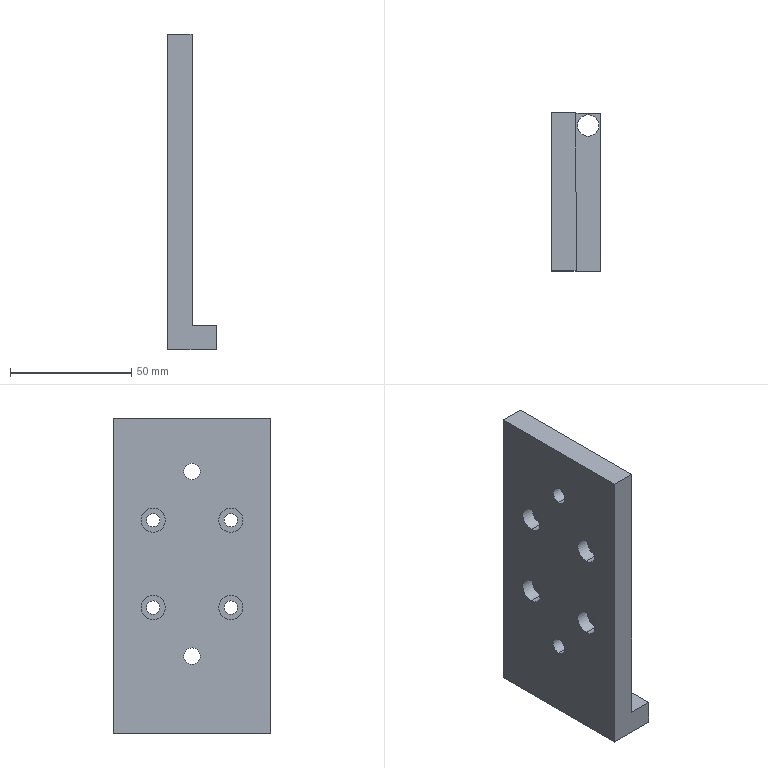Component | SolidWorks | SwingCylinderMountingPlate-1 | 1 solid | 34 faces | box 20.01 x 65 x 130 mm | volume 87532 mm3 | cylinder 22 | plane 12 | commonest cylinder face diameters 10 x8 5.5 x8 6.8 x4 8.8 x2
build123d program:
from build123d import *

# Parameters (mm, degrees)
SKETCH1_W                                       = 120
SKETCH1_H                                       = 65
BOSS_EXTRUDE1_DEPTH                             = 10
M8_TAPPED_HOLE1_D                               = 6.8
M8_TAPPED_HOLE1_DEPTH                           = 19.75
M8_TAPPED_HOLE1_TIP                             = 2.043
M5_HEX_SOCKET_HEAD_CAP_SCREW_CBORE1_D           = 5.5
M5_HEX_SOCKET_HEAD_CAP_SCREW_CBORE1_DEPTH       = 19.75
M5_HEX_SOCKET_HEAD_CAP_SCREW_CBORE1_CBORE_D     = 10
M5_HEX_SOCKET_HEAD_CAP_SCREW_CBORE1_CBORE_DEPTH = 5.4
M5_HEX_SOCKET_HEAD_CAP_SCREW_CBORE1_TIP         = 1.652
SKETCH6_W                                       = 20
SKETCH6_H                                       = 65
BOSS_EXTRUDE2_DEPTH                             = 10
M10X1_25_TAPPED_HOLE1_D                         = 8.8
M10X1_25_TAPPED_HOLE1_DEPTH                     = 23.75
M10X1_25_TAPPED_HOLE1_TIP                       = 2.644


with BuildPart() as part:
    # Sketch1 → Boss-Extrude1 (new body)
    with BuildSketch(Plane.XY):
        Rectangle(SKETCH1_W, SKETCH1_H)
    extrude(amount=BOSS_EXTRUDE1_DEPTH)

    # M8 Tapped Hole1
    with Locations(Plane.XY.offset(10)):
        with Locations((-38, 0), (38, 0)):
            Hole(M8_TAPPED_HOLE1_D / 2, depth=M8_TAPPED_HOLE1_DEPTH)
            with Locations((0, 0, -(M8_TAPPED_HOLE1_DEPTH + M8_TAPPED_HOLE1_TIP / 2))):  # 118° drill point
                Cone(0, M8_TAPPED_HOLE1_D / 2, M8_TAPPED_HOLE1_TIP, mode=Mode.SUBTRACT)

    # M5 Hex Socket Head Cap Screw CBORE1
    with Locations(Plane.XY.offset(10)):
        with Locations((-18, 16), (18, 16), (-18, -16), (18, -16)):
            CounterBoreHole(M5_HEX_SOCKET_HEAD_CAP_SCREW_CBORE1_D / 2, M5_HEX_SOCKET_HEAD_CAP_SCREW_CBORE1_CBORE_D / 2, M5_HEX_SOCKET_HEAD_CAP_SCREW_CBORE1_CBORE_DEPTH, depth=M5_HEX_SOCKET_HEAD_CAP_SCREW_CBORE1_DEPTH)
            with Locations((0, 0, -(M5_HEX_SOCKET_HEAD_CAP_SCREW_CBORE1_DEPTH + M5_HEX_SOCKET_HEAD_CAP_SCREW_CBORE1_TIP / 2))):  # 118° drill point
                Cone(0, M5_HEX_SOCKET_HEAD_CAP_SCREW_CBORE1_D / 2, M5_HEX_SOCKET_HEAD_CAP_SCREW_CBORE1_TIP, mode=Mode.SUBTRACT)

    # Sketch6 → Boss-Extrude2 (add)
    with BuildSketch(Plane.ZY.offset(60)):
        Rectangle(SKETCH6_W, SKETCH6_H)
    extrude(amount=BOSS_EXTRUDE2_DEPTH)

    # M10x1.25 Tapped Hole1
    with Locations(Plane.ZY.offset(70)):
        with Locations((-5, 27.5)):
            Hole(M10X1_25_TAPPED_HOLE1_D / 2, depth=M10X1_25_TAPPED_HOLE1_DEPTH)
            with Locations((0, 0, -(M10X1_25_TAPPED_HOLE1_DEPTH + M10X1_25_TAPPED_HOLE1_TIP / 2))):  # 118° drill point
                Cone(0, M10X1_25_TAPPED_HOLE1_D / 2, M10X1_25_TAPPED_HOLE1_TIP, mode=Mode.SUBTRACT)


solid = part.part

# Placed as in the assembly
solid = solid.moved(Location((1956.163, 3833.759, 1079.241), (0, -90, 0)))
STEP:
#1=CARTESIAN_POINT('',(77.038,152.018,40.128));
#2=VERTEX_POINT('',#1);
#3=CARTESIAN_POINT('',(77.384,152.018,40.128));
#4=VERTEX_POINT('',#3);
#5=CARTESIAN_POINT('',(77.211,152.018,40.128));
#6=DIRECTION('',(-0.,-0.,1.));
#7=DIRECTION('',(1.,0.0001552,0.));
#8=AXIS2_PLACEMENT_3D('',#5,#6,#7);
#9=CIRCLE('',#8,0.1732);
#10=EDGE_CURVE('',#2,#4,#9,.T.);
#11=ORIENTED_EDGE('',*,*,#10,.T.);
#12=CARTESIAN_POINT('',(77.384,152.018,39.734));
#13=VERTEX_POINT('',#12);
#14=CARTESIAN_POINT('',(77.384,152.018,39.734));
#15=DIRECTION('',(0.,0.,-1.));
#16=VECTOR('',#15,39.37);
#17=LINE('',#14,#16);
#18=EDGE_CURVE('',#4,#13,#17,.T.);
#19=ORIENTED_EDGE('',*,*,#18,.T.);
#20=CARTESIAN_POINT('',(77.038,152.018,39.734));
#21=VERTEX_POINT('',#20);
#22=CARTESIAN_POINT('',(77.211,152.018,39.734));
#23=DIRECTION('',(0.,0.,-1.));
#24=DIRECTION('',(-1.,-0.0001552,0.));
#25=AXIS2_PLACEMENT_3D('',#22,#23,#24);
#26=CIRCLE('',#25,0.1732);
#27=EDGE_CURVE('',#13,#21,#26,.T.);
#28=ORIENTED_EDGE('',*,*,#27,.T.);
#29=CARTESIAN_POINT('',(77.038,152.018,39.734));
#30=DIRECTION('',(0.,0.,-1.));
#31=VECTOR('',#30,39.37);
#32=LINE('',#29,#31);
#33=EDGE_CURVE('',#2,#21,#32,.T.);
#34=ORIENTED_EDGE('',*,*,#33,.F.);
#35=EDGE_LOOP('',(#11,#19,#28,#34));
#36=FACE_OUTER_BOUND('',#35,.T.);
#37=CARTESIAN_POINT('',(77.211,152.018,39.734));
#38=DIRECTION('',(0.,0.,-1.));
#39=DIRECTION('',(-1.,-0.0001552,0.));
#40=AXIS2_PLACEMENT_3D('',#37,#38,#39);
#41=CYLINDRICAL_SURFACE('',#40,0.1732);
#42=ADVANCED_FACE('',(#36),#41,.F.);
#43=CARTESIAN_POINT('',(76.833,151.565,41.584));
#44=VERTEX_POINT('',#43);
#45=CARTESIAN_POINT('',(76.833,151.565,41.978));
#46=VERTEX_POINT('',#45);
#47=CARTESIAN_POINT('',(76.833,151.565,41.781));
#48=DIRECTION('',(-1.,-0.0001552,-0.));
#49=DIRECTION('',(0.,0.,1.));
#50=AXIS2_PLACEMENT_3D('',#47,#48,#49);
#51=CIRCLE('',#50,0.1969);
#52=EDGE_CURVE('',#44,#46,#51,.T.);
#53=ORIENTED_EDGE('',*,*,#52,.F.);
#54=CARTESIAN_POINT('',(76.621,151.565,41.584));
#55=VERTEX_POINT('',#54);
#56=CARTESIAN_POINT('',(76.621,151.565,41.584));
#57=DIRECTION('',(-1.,-0.0001552,-0.));
#58=VECTOR('',#57,39.37);
#59=LINE('',#56,#58);
#60=EDGE_CURVE('',#44,#55,#59,.T.);
#61=ORIENTED_EDGE('',*,*,#60,.T.);
#62=CARTESIAN_POINT('',(76.621,151.565,41.978));
#63=VERTEX_POINT('',#62);
#64=CARTESIAN_POINT('',(76.621,151.565,41.781));
#65=DIRECTION('',(-1.,-0.0001552,-0.));
#66=DIRECTION('',(0.,0.,1.));
#67=AXIS2_PLACEMENT_3D('',#64,#65,#66);
#68=CIRCLE('',#67,0.1969);
#69=EDGE_CURVE('',#55,#63,#68,.T.);
#70=ORIENTED_EDGE('',*,*,#69,.T.);
#71=CARTESIAN_POINT('',(76.621,151.565,41.978));
#72=DIRECTION('',(-1.,-0.0001552,-0.));
#73=VECTOR('',#72,39.37);
#74=LINE('',#71,#73);
#75=EDGE_CURVE('',#46,#63,#74,.T.);
#76=ORIENTED_EDGE('',*,*,#75,.F.);
#77=EDGE_LOOP('',(#53,#61,#70,#76));
#78=FACE_OUTER_BOUND('',#77,.T.);
#79=CARTESIAN_POINT('',(76.621,151.565,41.781));
#80=DIRECTION('',(-1.,-0.0001552,-0.));
#81=DIRECTION('',(0.,0.,1.));
#82=AXIS2_PLACEMENT_3D('',#79,#80,#81);
#83=CYLINDRICAL_SURFACE('',#82,0.1969);
#84=ADVANCED_FACE('',(#78),#83,.F.);
#85=CARTESIAN_POINT('',(77.014,151.565,41.673));
#86=VERTEX_POINT('',#85);
#87=CARTESIAN_POINT('',(77.014,151.565,41.889));
#88=VERTEX_POINT('',#87);
#89=CARTESIAN_POINT('',(77.014,151.565,41.781));
#90=DIRECTION('',(-1.,-0.0001552,-0.));
#91=DIRECTION('',(0.,0.,1.));
#92=AXIS2_PLACEMENT_3D('',#89,#90,#91);
#93=CIRCLE('',#92,0.1083);
#94=EDGE_CURVE('',#86,#88,#93,.T.);
#95=ORIENTED_EDGE('',*,*,#94,.F.);
#96=CARTESIAN_POINT('',(76.833,151.565,41.673));
#97=VERTEX_POINT('',#96);
#98=CARTESIAN_POINT('',(76.621,151.565,41.673));
#99=DIRECTION('',(-1.,-0.0001552,-0.));
#100=VECTOR('',#99,39.37);
#101=LINE('',#98,#100);
#102=EDGE_CURVE('',#86,#97,#101,.T.);
#103=ORIENTED_EDGE('',*,*,#102,.T.);
#104=CARTESIAN_POINT('',(76.833,151.565,41.889));
#105=VERTEX_POINT('',#104);
#106=CARTESIAN_POINT('',(76.833,151.565,41.781));
#107=DIRECTION('',(-1.,-0.0001552,-0.));
#108=DIRECTION('',(0.,0.,1.));
#109=AXIS2_PLACEMENT_3D('',#106,#107,#108);
#110=CIRCLE('',#109,0.1083);
#111=EDGE_CURVE('',#97,#105,#110,.T.);
#112=ORIENTED_EDGE('',*,*,#111,.T.);
#113=CARTESIAN_POINT('',(76.621,151.565,41.889));
#114=DIRECTION('',(-1.,-0.0001552,-0.));
#115=VECTOR('',#114,39.37);
#116=LINE('',#113,#115);
#117=EDGE_CURVE('',#88,#105,#116,.T.);
#118=ORIENTED_EDGE('',*,*,#117,.F.);
#119=EDGE_LOOP('',(#95,#103,#112,#118));
#120=FACE_OUTER_BOUND('',#119,.T.);
#121=CARTESIAN_POINT('',(76.621,151.565,41.781));
#122=DIRECTION('',(-1.,-0.0001552,-0.));
#123=DIRECTION('',(0.,0.,1.));
#124=AXIS2_PLACEMENT_3D('',#121,#122,#123);
#125=CYLINDRICAL_SURFACE('',#124,0.1083);
#126=ADVANCED_FACE('',(#120),#125,.F.);
#127=CARTESIAN_POINT('',(76.833,151.565,43.002));
#128=VERTEX_POINT('',#127);
#129=CARTESIAN_POINT('',(76.833,151.565,43.395));
#130=VERTEX_POINT('',#129);
#131=CARTESIAN_POINT('',(76.833,151.565,43.198));
#132=DIRECTION('',(-1.,-0.0001552,-0.));
#133=DIRECTION('',(0.,0.,1.));
#134=AXIS2_PLACEMENT_3D('',#131,#132,#133);
#135=CIRCLE('',#134,0.1969);
#136=EDGE_CURVE('',#128,#130,#135,.T.);
#137=ORIENTED_EDGE('',*,*,#136,.F.);
#138=CARTESIAN_POINT('',(76.621,151.565,43.002));
#139=VERTEX_POINT('',#138);
#140=CARTESIAN_POINT('',(76.621,151.565,43.002));
#141=DIRECTION('',(-1.,-0.0001552,-0.));
#142=VECTOR('',#141,39.37);
#143=LINE('',#140,#142);
#144=EDGE_CURVE('',#128,#139,#143,.T.);
#145=ORIENTED_EDGE('',*,*,#144,.T.);
#146=CARTESIAN_POINT('',(76.621,151.565,43.395));
#147=VERTEX_POINT('',#146);
#148=CARTESIAN_POINT('',(76.621,151.565,43.198));
#149=DIRECTION('',(-1.,-0.0001552,-0.));
#150=DIRECTION('',(0.,0.,1.));
#151=AXIS2_PLACEMENT_3D('',#148,#149,#150);
#152=CIRCLE('',#151,0.1969);
#153=EDGE_CURVE('',#139,#147,#152,.T.);
#154=ORIENTED_EDGE('',*,*,#153,.T.);
#155=CARTESIAN_POINT('',(76.621,151.565,43.395));
#156=DIRECTION('',(-1.,-0.0001552,-0.));
#157=VECTOR('',#156,39.37);
#158=LINE('',#155,#157);
#159=EDGE_CURVE('',#130,#147,#158,.T.);
#160=ORIENTED_EDGE('',*,*,#159,.F.);
#161=EDGE_LOOP('',(#137,#145,#154,#160));
#162=FACE_OUTER_BOUND('',#161,.T.);
#163=CARTESIAN_POINT('',(76.621,151.565,43.198));
#164=DIRECTION('',(-1.,-0.0001552,-0.));
#165=DIRECTION('',(0.,0.,1.));
#166=AXIS2_PLACEMENT_3D('',#163,#164,#165);
#167=CYLINDRICAL_SURFACE('',#166,0.1969);
#168=ADVANCED_FACE('',(#162),#167,.F.);
#169=CARTESIAN_POINT('',(77.014,151.565,43.09));
#170=VERTEX_POINT('',#169);
#171=CARTESIAN_POINT('',(77.014,151.565,43.307));
#172=VERTEX_POINT('',#171);
#173=CARTESIAN_POINT('',(77.014,151.565,43.198));
#174=DIRECTION('',(-1.,-0.0001552,-0.));
#175=DIRECTION('',(0.,0.,1.));
#176=AXIS2_PLACEMENT_3D('',#173,#174,#175);
#177=CIRCLE('',#176,0.1083);
#178=EDGE_CURVE('',#170,#172,#177,.T.);
#179=ORIENTED_EDGE('',*,*,#178,.F.);
#180=CARTESIAN_POINT('',(76.833,151.565,43.09));
#181=VERTEX_POINT('',#180);
#182=CARTESIAN_POINT('',(76.621,151.565,43.09));
#183=DIRECTION('',(-1.,-0.0001552,-0.));
#184=VECTOR('',#183,39.37);
#185=LINE('',#182,#184);
#186=EDGE_CURVE('',#170,#181,#185,.T.);
#187=ORIENTED_EDGE('',*,*,#186,.T.);
#188=CARTESIAN_POINT('',(76.833,151.565,43.307));
#189=VERTEX_POINT('',#188);
#190=CARTESIAN_POINT('',(76.833,151.565,43.198));
#191=DIRECTION('',(-1.,-0.0001552,-0.));
#192=DIRECTION('',(0.,0.,1.));
#193=AXIS2_PLACEMENT_3D('',#190,#191,#192);
#194=CIRCLE('',#193,0.1083);
#195=EDGE_CURVE('',#181,#189,#194,.T.);
#196=ORIENTED_EDGE('',*,*,#195,.T.);
#197=CARTESIAN_POINT('',(76.621,151.565,43.307));
#198=DIRECTION('',(-1.,-0.0001552,-0.));
#199=VECTOR('',#198,39.37);
#200=LINE('',#197,#199);
#201=EDGE_CURVE('',#172,#189,#200,.T.);
#202=ORIENTED_EDGE('',*,*,#201,.F.);
#203=EDGE_LOOP('',(#179,#187,#196,#202));
#204=FACE_OUTER_BOUND('',#203,.T.);
#205=CARTESIAN_POINT('',(76.621,151.565,43.198));
#206=DIRECTION('',(-1.,-0.0001552,-0.));
#207=DIRECTION('',(0.,0.,1.));
#208=AXIS2_PLACEMENT_3D('',#205,#206,#207);
#209=CYLINDRICAL_SURFACE('',#208,0.1083);
#210=ADVANCED_FACE('',(#204),#209,.F.);
#211=CARTESIAN_POINT('',(76.833,150.305,41.584));
#212=VERTEX_POINT('',#211);
#213=CARTESIAN_POINT('',(76.833,150.305,41.978));
#214=VERTEX_POINT('',#213);
#215=CARTESIAN_POINT('',(76.833,150.305,41.781));
#216=DIRECTION('',(-1.,-0.0001552,-0.));
#217=DIRECTION('',(0.,0.,1.));
#218=AXIS2_PLACEMENT_3D('',#215,#216,#217);
#219=CIRCLE('',#218,0.1969);
#220=EDGE_CURVE('',#212,#214,#219,.T.);
#221=ORIENTED_EDGE('',*,*,#220,.F.);
#222=CARTESIAN_POINT('',(76.621,150.305,41.584));
#223=VERTEX_POINT('',#222);
#224=CARTESIAN_POINT('',(76.621,150.305,41.584));
#225=DIRECTION('',(-1.,-0.0001552,-0.));
#226=VECTOR('',#225,39.37);
#227=LINE('',#224,#226);
#228=EDGE_CURVE('',#212,#223,#227,.T.);
#229=ORIENTED_EDGE('',*,*,#228,.T.);
#230=CARTESIAN_POINT('',(76.621,150.305,41.978));
#231=VERTEX_POINT('',#230);
#232=CARTESIAN_POINT('',(76.621,150.305,41.781));
#233=DIRECTION('',(-1.,-0.0001552,-0.));
#234=DIRECTION('',(0.,0.,1.));
#235=AXIS2_PLACEMENT_3D('',#232,#233,#234);
#236=CIRCLE('',#235,0.1969);
#237=EDGE_CURVE('',#223,#231,#236,.T.);
#238=ORIENTED_EDGE('',*,*,#237,.T.);
#239=CARTESIAN_POINT('',(76.621,150.305,41.978));
#240=DIRECTION('',(-1.,-0.0001552,-0.));
#241=VECTOR('',#240,39.37);
#242=LINE('',#239,#241);
#243=EDGE_CURVE('',#214,#231,#242,.T.);
#244=ORIENTED_EDGE('',*,*,#243,.F.);
#245=EDGE_LOOP('',(#221,#229,#238,#244));
#246=FACE_OUTER_BOUND('',#245,.T.);
#247=CARTESIAN_POINT('',(76.621,150.305,41.781));
#248=DIRECTION('',(-1.,-0.0001552,-0.));
#249=DIRECTION('',(0.,0.,1.));
#250=AXIS2_PLACEMENT_3D('',#247,#248,#249);
#251=CYLINDRICAL_SURFACE('',#250,0.1969);
#252=ADVANCED_FACE('',(#246),#251,.F.);
#253=CARTESIAN_POINT('',(77.014,150.305,41.673));
#254=VERTEX_POINT('',#253);
#255=CARTESIAN_POINT('',(77.014,150.305,41.889));
#256=VERTEX_POINT('',#255);
#257=CARTESIAN_POINT('',(77.014,150.305,41.781));
#258=DIRECTION('',(-1.,-0.0001552,-0.));
#259=DIRECTION('',(0.,0.,1.));
#260=AXIS2_PLACEMENT_3D('',#257,#258,#259);
#261=CIRCLE('',#260,0.1083);
#262=EDGE_CURVE('',#254,#256,#261,.T.);
#263=ORIENTED_EDGE('',*,*,#262,.F.);
#264=CARTESIAN_POINT('',(76.833,150.305,41.673));
#265=VERTEX_POINT('',#264);
#266=CARTESIAN_POINT('',(76.621,150.305,41.673));
#267=DIRECTION('',(-1.,-0.0001552,-0.));
#268=VECTOR('',#267,39.37);
#269=LINE('',#266,#268);
#270=EDGE_CURVE('',#254,#265,#269,.T.);
#271=ORIENTED_EDGE('',*,*,#270,.T.);
#272=CARTESIAN_POINT('',(76.833,150.305,41.889));
#273=VERTEX_POINT('',#272);
#274=CARTESIAN_POINT('',(76.833,150.305,41.781));
#275=DIRECTION('',(-1.,-0.0001552,-0.));
#276=DIRECTION('',(0.,0.,1.));
#277=AXIS2_PLACEMENT_3D('',#274,#275,#276);
#278=CIRCLE('',#277,0.1083);
#279=EDGE_CURVE('',#265,#273,#278,.T.);
#280=ORIENTED_EDGE('',*,*,#279,.T.);
#281=CARTESIAN_POINT('',(76.621,150.305,41.889));
#282=DIRECTION('',(-1.,-0.0001552,-0.));
#283=VECTOR('',#282,39.37);
#284=LINE('',#281,#283);
#285=EDGE_CURVE('',#256,#273,#284,.T.);
#286=ORIENTED_EDGE('',*,*,#285,.F.);
#287=EDGE_LOOP('',(#263,#271,#280,#286));
#288=FACE_OUTER_BOUND('',#287,.T.);
#289=CARTESIAN_POINT('',(76.621,150.305,41.781));
#290=DIRECTION('',(-1.,-0.0001552,-0.));
#291=DIRECTION('',(0.,0.,1.));
#292=AXIS2_PLACEMENT_3D('',#289,#290,#291);
#293=CYLINDRICAL_SURFACE('',#292,0.1083);
#294=ADVANCED_FACE('',(#288),#293,.F.);
#295=CARTESIAN_POINT('',(76.833,150.305,43.002));
#296=VERTEX_POINT('',#295);
#297=CARTESIAN_POINT('',(76.833,150.305,43.395));
#298=VERTEX_POINT('',#297);
#299=CARTESIAN_POINT('',(76.833,150.305,43.198));
#300=DIRECTION('',(-1.,-0.0001552,-0.));
#301=DIRECTION('',(0.,0.,1.));
#302=AXIS2_PLACEMENT_3D('',#299,#300,#301);
#303=CIRCLE('',#302,0.1969);
#304=EDGE_CURVE('',#296,#298,#303,.T.);
#305=ORIENTED_EDGE('',*,*,#304,.F.);
#306=CARTESIAN_POINT('',(76.621,150.305,43.002));
#307=VERTEX_POINT('',#306);
#308=CARTESIAN_POINT('',(76.621,150.305,43.002));
#309=DIRECTION('',(-1.,-0.0001552,-0.));
#310=VECTOR('',#309,39.37);
#311=LINE('',#308,#310);
#312=EDGE_CURVE('',#296,#307,#311,.T.);
#313=ORIENTED_EDGE('',*,*,#312,.T.);
#314=CARTESIAN_POINT('',(76.621,150.305,43.395));
#315=VERTEX_POINT('',#314);
#316=CARTESIAN_POINT('',(76.621,150.305,43.198));
#317=DIRECTION('',(-1.,-0.0001552,-0.));
#318=DIRECTION('',(0.,0.,1.));
#319=AXIS2_PLACEMENT_3D('',#316,#317,#318);
#320=CIRCLE('',#319,0.1969);
#321=EDGE_CURVE('',#307,#315,#320,.T.);
#322=ORIENTED_EDGE('',*,*,#321,.T.);
#323=CARTESIAN_POINT('',(76.621,150.305,43.395));
#324=DIRECTION('',(-1.,-0.0001552,-0.));
#325=VECTOR('',#324,39.37);
#326=LINE('',#323,#325);
#327=EDGE_CURVE('',#298,#315,#326,.T.);
#328=ORIENTED_EDGE('',*,*,#327,.F.);
#329=EDGE_LOOP('',(#305,#313,#322,#328));
#330=FACE_OUTER_BOUND('',#329,.T.);
#331=CARTESIAN_POINT('',(76.621,150.305,43.198));
#332=DIRECTION('',(-1.,-0.0001552,-0.));
#333=DIRECTION('',(0.,0.,1.));
#334=AXIS2_PLACEMENT_3D('',#331,#332,#333);
#335=CYLINDRICAL_SURFACE('',#334,0.1969);
#336=ADVANCED_FACE('',(#330),#335,.F.);
#337=CARTESIAN_POINT('',(77.014,150.305,43.09));
#338=VERTEX_POINT('',#337);
#339=CARTESIAN_POINT('',(77.014,150.305,43.307));
#340=VERTEX_POINT('',#339);
#341=CARTESIAN_POINT('',(77.014,150.305,43.198));
#342=DIRECTION('',(-1.,-0.0001552,-0.));
#343=DIRECTION('',(0.,0.,1.));
#344=AXIS2_PLACEMENT_3D('',#341,#342,#343);
#345=CIRCLE('',#344,0.1083);
#346=EDGE_CURVE('',#338,#340,#345,.T.);
#347=ORIENTED_EDGE('',*,*,#346,.F.);
#348=CARTESIAN_POINT('',(76.833,150.305,43.09));
#349=VERTEX_POINT('',#348);
#350=CARTESIAN_POINT('',(76.621,150.305,43.09));
#351=DIRECTION('',(-1.,-0.0001552,-0.));
#352=VECTOR('',#351,39.37);
#353=LINE('',#350,#352);
#354=EDGE_CURVE('',#338,#349,#353,.T.);
#355=ORIENTED_EDGE('',*,*,#354,.T.);
#356=CARTESIAN_POINT('',(76.833,150.305,43.307));
#357=VERTEX_POINT('',#356);
#358=CARTESIAN_POINT('',(76.833,150.305,43.198));
#359=DIRECTION('',(-1.,-0.0001552,-0.));
#360=DIRECTION('',(0.,0.,1.));
#361=AXIS2_PLACEMENT_3D('',#358,#359,#360);
#362=CIRCLE('',#361,0.1083);
#363=EDGE_CURVE('',#349,#357,#362,.T.);
#364=ORIENTED_EDGE('',*,*,#363,.T.);
#365=CARTESIAN_POINT('',(76.621,150.305,43.307));
#366=DIRECTION('',(-1.,-0.0001552,-0.));
#367=VECTOR('',#366,39.37);
#368=LINE('',#365,#367);
#369=EDGE_CURVE('',#340,#357,#368,.T.);
#370=ORIENTED_EDGE('',*,*,#369,.F.);
#371=EDGE_LOOP('',(#347,#355,#364,#370));
#372=FACE_OUTER_BOUND('',#371,.T.);
#373=CARTESIAN_POINT('',(76.621,150.305,43.198));
#374=DIRECTION('',(-1.,-0.0001552,-0.));
#375=DIRECTION('',(0.,0.,1.));
#376=AXIS2_PLACEMENT_3D('',#373,#374,#375);
#377=CYLINDRICAL_SURFACE('',#376,0.1083);
#378=ADVANCED_FACE('',(#372),#377,.F.);
#379=CARTESIAN_POINT('',(77.014,150.935,40.86));
#380=VERTEX_POINT('',#379);
#381=CARTESIAN_POINT('',(77.014,150.935,41.128));
#382=VERTEX_POINT('',#381);
#383=CARTESIAN_POINT('',(77.014,150.935,40.994));
#384=DIRECTION('',(-1.,-0.0001552,-0.));
#385=DIRECTION('',(0.,0.,1.));
#386=AXIS2_PLACEMENT_3D('',#383,#384,#385);
#387=CIRCLE('',#386,0.1339);
#388=EDGE_CURVE('',#380,#382,#387,.T.);
#389=ORIENTED_EDGE('',*,*,#388,.F.);
#390=CARTESIAN_POINT('',(76.621,150.935,40.86));
#391=VERTEX_POINT('',#390);
#392=CARTESIAN_POINT('',(76.621,150.935,40.86));
#393=DIRECTION('',(-1.,-0.0001552,-0.));
#394=VECTOR('',#393,39.37);
#395=LINE('',#392,#394);
#396=EDGE_CURVE('',#380,#391,#395,.T.);
#397=ORIENTED_EDGE('',*,*,#396,.T.);
#398=CARTESIAN_POINT('',(76.621,150.935,41.128));
#399=VERTEX_POINT('',#398);
#400=CARTESIAN_POINT('',(76.621,150.935,40.994));
#401=DIRECTION('',(-1.,-0.0001552,-0.));
#402=DIRECTION('',(0.,0.,1.));
#403=AXIS2_PLACEMENT_3D('',#400,#401,#402);
#404=CIRCLE('',#403,0.1339);
#405=EDGE_CURVE('',#391,#399,#404,.T.);
#406=ORIENTED_EDGE('',*,*,#405,.T.);
#407=CARTESIAN_POINT('',(76.621,150.935,41.128));
#408=DIRECTION('',(-1.,-0.0001552,-0.));
#409=VECTOR('',#408,39.37);
#410=LINE('',#407,#409);
#411=EDGE_CURVE('',#382,#399,#410,.T.);
#412=ORIENTED_EDGE('',*,*,#411,.F.);
#413=EDGE_LOOP('',(#389,#397,#406,#412));
#414=FACE_OUTER_BOUND('',#413,.T.);
#415=CARTESIAN_POINT('',(76.621,150.935,40.994));
#416=DIRECTION('',(-1.,-0.0001552,-0.));
#417=DIRECTION('',(0.,0.,1.));
#418=AXIS2_PLACEMENT_3D('',#415,#416,#417);
#419=CYLINDRICAL_SURFACE('',#418,0.1339);
#420=ADVANCED_FACE('',(#414),#419,.F.);
#421=CARTESIAN_POINT('',(77.014,150.935,43.852));
#422=VERTEX_POINT('',#421);
#423=CARTESIAN_POINT('',(77.014,150.935,44.12));
#424=VERTEX_POINT('',#423);
#425=CARTESIAN_POINT('',(77.014,150.935,43.986));
#426=DIRECTION('',(-1.,-0.0001552,-0.));
#427=DIRECTION('',(0.,0.,1.));
#428=AXIS2_PLACEMENT_3D('',#425,#426,#427);
#429=CIRCLE('',#428,0.1339);
#430=EDGE_CURVE('',#422,#424,#429,.T.);
#431=ORIENTED_EDGE('',*,*,#430,.F.);
#432=CARTESIAN_POINT('',(76.621,150.935,43.852));
#433=VERTEX_POINT('',#432);
#434=CARTESIAN_POINT('',(76.621,150.935,43.852));
#435=DIRECTION('',(-1.,-0.0001552,-0.));
#436=VECTOR('',#435,39.37);
#437=LINE('',#434,#436);
#438=EDGE_CURVE('',#422,#433,#437,.T.);
#439=ORIENTED_EDGE('',*,*,#438,.T.);
#440=CARTESIAN_POINT('',(76.621,150.935,44.12));
#441=VERTEX_POINT('',#440);
#442=CARTESIAN_POINT('',(76.621,150.935,43.986));
#443=DIRECTION('',(-1.,-0.0001552,-0.));
#444=DIRECTION('',(0.,0.,1.));
#445=AXIS2_PLACEMENT_3D('',#442,#443,#444);
#446=CIRCLE('',#445,0.1339);
#447=EDGE_CURVE('',#433,#441,#446,.T.);
#448=ORIENTED_EDGE('',*,*,#447,.T.);
#449=CARTESIAN_POINT('',(76.621,150.935,44.12));
#450=DIRECTION('',(-1.,-0.0001552,-0.));
#451=VECTOR('',#450,39.37);
#452=LINE('',#449,#451);
#453=EDGE_CURVE('',#424,#441,#452,.T.);
#454=ORIENTED_EDGE('',*,*,#453,.F.);
#455=EDGE_LOOP('',(#431,#439,#448,#454));
#456=FACE_OUTER_BOUND('',#455,.T.);
#457=CARTESIAN_POINT('',(76.621,150.935,43.986));
#458=DIRECTION('',(-1.,-0.0001552,-0.));
#459=DIRECTION('',(0.,0.,1.));
#460=AXIS2_PLACEMENT_3D('',#457,#458,#459);
#461=CYLINDRICAL_SURFACE('',#460,0.1339);
#462=ADVANCED_FACE('',(#456),#461,.F.);
#463=CARTESIAN_POINT('',(77.015,149.656,40.128));
#464=VERTEX_POINT('',#463);
#465=CARTESIAN_POINT('',(77.015,149.656,44.852));
#466=VERTEX_POINT('',#465);
#467=CARTESIAN_POINT('',(77.015,149.656,44.852));
#468=DIRECTION('',(-0.,-0.,1.));
#469=VECTOR('',#468,39.37);
#470=LINE('',#467,#469);
#471=EDGE_CURVE('',#464,#466,#470,.T.);
#472=ORIENTED_EDGE('',*,*,#471,.T.);
#473=CARTESIAN_POINT('',(76.621,149.656,44.852));
#474=VERTEX_POINT('',#473);
#475=CARTESIAN_POINT('',(76.621,149.656,44.852));
#476=DIRECTION('',(1.,0.0001552,0.));
#477=VECTOR('',#476,39.37);
#478=LINE('',#475,#477);
#479=EDGE_CURVE('',#474,#466,#478,.T.);
#480=ORIENTED_EDGE('',*,*,#479,.F.);
#481=CARTESIAN_POINT('',(76.621,149.656,39.734));
#482=VERTEX_POINT('',#481);
#483=CARTESIAN_POINT('',(76.621,149.656,44.852));
#484=DIRECTION('',(-0.,-0.,1.));
#485=VECTOR('',#484,39.37);
#486=LINE('',#483,#485);
#487=EDGE_CURVE('',#482,#474,#486,.T.);
#488=ORIENTED_EDGE('',*,*,#487,.F.);
#489=CARTESIAN_POINT('',(77.408,149.656,39.734));
#490=VERTEX_POINT('',#489);
#491=CARTESIAN_POINT('',(76.621,149.656,39.734));
#492=DIRECTION('',(-1.,-0.0001552,-0.));
#493=VECTOR('',#492,39.37);
#494=LINE('',#491,#493);
#495=EDGE_CURVE('',#490,#482,#494,.T.);
#496=ORIENTED_EDGE('',*,*,#495,.F.);
#497=CARTESIAN_POINT('',(77.408,149.656,40.128));
#498=VERTEX_POINT('',#497);
#499=CARTESIAN_POINT('',(77.408,149.656,39.734));
#500=DIRECTION('',(-0.,-0.,1.));
#501=VECTOR('',#500,39.37);
#502=LINE('',#499,#501);
#503=EDGE_CURVE('',#490,#498,#502,.T.);
#504=ORIENTED_EDGE('',*,*,#503,.T.);
#505=CARTESIAN_POINT('',(76.621,149.656,40.128));
#506=DIRECTION('',(-1.,-0.0001552,-0.));
#507=VECTOR('',#506,39.37);
#508=LINE('',#505,#507);
#509=EDGE_CURVE('',#498,#464,#508,.T.);
#510=ORIENTED_EDGE('',*,*,#509,.T.);
#511=EDGE_LOOP('',(#472,#480,#488,#496,#504,#510));
#512=FACE_OUTER_BOUND('',#511,.T.);
#513=CARTESIAN_POINT('',(76.621,149.656,44.852));
#514=DIRECTION('',(-0.0001552,1.,0.));
#515=DIRECTION('',(0.,0.,-1.));
#516=AXIS2_PLACEMENT_3D('',#513,#514,#515);
#517=PLANE('',#516);
#518=ADVANCED_FACE('',(#512),#517,.F.);
#519=CARTESIAN_POINT('',(77.014,152.215,44.852));
#520=VERTEX_POINT('',#519);
#521=CARTESIAN_POINT('',(77.015,149.656,44.852));
#522=DIRECTION('',(-0.0001552,1.,0.));
#523=VECTOR('',#522,39.37);
#524=LINE('',#521,#523);
#525=EDGE_CURVE('',#466,#520,#524,.T.);
#526=ORIENTED_EDGE('',*,*,#525,.T.);
#527=CARTESIAN_POINT('',(76.62,152.215,44.852));
#528=VERTEX_POINT('',#527);
#529=CARTESIAN_POINT('',(76.62,152.215,44.852));
#530=DIRECTION('',(1.,0.0001552,0.));
#531=VECTOR('',#530,39.37);
#532=LINE('',#529,#531);
#533=EDGE_CURVE('',#528,#520,#532,.T.);
#534=ORIENTED_EDGE('',*,*,#533,.F.);
#535=CARTESIAN_POINT('',(76.621,149.656,44.852));
#536=DIRECTION('',(-0.0001552,1.,0.));
#537=VECTOR('',#536,39.37);
#538=LINE('',#535,#537);
#539=EDGE_CURVE('',#474,#528,#538,.T.);
#540=ORIENTED_EDGE('',*,*,#539,.F.);
#541=ORIENTED_EDGE('',*,*,#479,.T.);
#542=EDGE_LOOP('',(#526,#534,#540,#541));
#543=FACE_OUTER_BOUND('',#542,.T.);
#544=CARTESIAN_POINT('',(76.621,149.656,44.852));
#545=DIRECTION('',(0.,0.,-1.));
#546=DIRECTION('',(-1.,-0.0001552,-0.));
#547=AXIS2_PLACEMENT_3D('',#544,#545,#546);
#548=PLANE('',#547);
#549=ADVANCED_FACE('',(#543),#548,.F.);
#550=CARTESIAN_POINT('',(77.014,152.215,40.128));
#551=VERTEX_POINT('',#550);
#552=CARTESIAN_POINT('',(77.014,152.215,44.852));
#553=DIRECTION('',(0.,0.,-1.));
#554=VECTOR('',#553,39.37);
#555=LINE('',#552,#554);
#556=EDGE_CURVE('',#520,#551,#555,.T.);
#557=ORIENTED_EDGE('',*,*,#556,.T.);
#558=CARTESIAN_POINT('',(77.408,152.215,40.128));
#559=VERTEX_POINT('',#558);
#560=CARTESIAN_POINT('',(76.62,152.215,40.128));
#561=DIRECTION('',(1.,0.0001552,0.));
#562=VECTOR('',#561,39.37);
#563=LINE('',#560,#562);
#564=EDGE_CURVE('',#551,#559,#563,.T.);
#565=ORIENTED_EDGE('',*,*,#564,.T.);
#566=CARTESIAN_POINT('',(77.408,152.215,39.734));
#567=VERTEX_POINT('',#566);
#568=CARTESIAN_POINT('',(77.408,152.215,39.734));
#569=DIRECTION('',(-0.,-0.,1.));
#570=VECTOR('',#569,39.37);
#571=LINE('',#568,#570);
#572=EDGE_CURVE('',#567,#559,#571,.T.);
#573=ORIENTED_EDGE('',*,*,#572,.F.);
#574=CARTESIAN_POINT('',(76.62,152.215,39.734));
#575=VERTEX_POINT('',#574);
#576=CARTESIAN_POINT('',(76.62,152.215,39.734));
#577=DIRECTION('',(1.,0.0001552,0.));
#578=VECTOR('',#577,39.37);
#579=LINE('',#576,#578);
#580=EDGE_CURVE('',#575,#567,#579,.T.);
#581=ORIENTED_EDGE('',*,*,#580,.F.);
#582=CARTESIAN_POINT('',(76.62,152.215,44.852));
#583=DIRECTION('',(0.,0.,-1.));
#584=VECTOR('',#583,39.37);
#585=LINE('',#582,#584);
#586=EDGE_CURVE('',#528,#575,#585,.T.);
#587=ORIENTED_EDGE('',*,*,#586,.F.);
#588=ORIENTED_EDGE('',*,*,#533,.T.);
#589=EDGE_LOOP('',(#557,#565,#573,#581,#587,#588));
#590=FACE_OUTER_BOUND('',#589,.T.);
#591=CARTESIAN_POINT('',(76.62,152.215,44.852));
#592=DIRECTION('',(0.0001552,-1.,-0.));
#593=DIRECTION('',(-0.,-0.,1.));
#594=AXIS2_PLACEMENT_3D('',#591,#592,#593);
#595=PLANE('',#594);
#596=ADVANCED_FACE('',(#590),#595,.F.);
#597=CARTESIAN_POINT('',(76.621,151.565,41.781));
#598=DIRECTION('',(-1.,-0.0001552,-0.));
#599=DIRECTION('',(0.,0.,1.));
#600=AXIS2_PLACEMENT_3D('',#597,#598,#599);
#601=CIRCLE('',#600,0.1969);
#602=EDGE_CURVE('',#63,#55,#601,.T.);
#603=ORIENTED_EDGE('',*,*,#602,.F.);
#604=ORIENTED_EDGE('',*,*,#69,.F.);
#605=EDGE_LOOP('',(#603,#604));
#606=FACE_BOUND('',#605,.T.);
#607=CARTESIAN_POINT('',(76.621,151.565,43.198));
#608=DIRECTION('',(-1.,-0.0001552,-0.));
#609=DIRECTION('',(0.,0.,1.));
#610=AXIS2_PLACEMENT_3D('',#607,#608,#609);
#611=CIRCLE('',#610,0.1969);
#612=EDGE_CURVE('',#147,#139,#611,.T.);
#613=ORIENTED_EDGE('',*,*,#612,.F.);
#614=ORIENTED_EDGE('',*,*,#153,.F.);
#615=EDGE_LOOP('',(#613,#614));
#616=FACE_BOUND('',#615,.T.);
#617=CARTESIAN_POINT('',(76.621,150.305,41.781));
#618=DIRECTION('',(-1.,-0.0001552,-0.));
#619=DIRECTION('',(0.,0.,1.));
#620=AXIS2_PLACEMENT_3D('',#617,#618,#619);
#621=CIRCLE('',#620,0.1969);
#622=EDGE_CURVE('',#231,#223,#621,.T.);
#623=ORIENTED_EDGE('',*,*,#622,.F.);
#624=ORIENTED_EDGE('',*,*,#237,.F.);
#625=EDGE_LOOP('',(#623,#624));
#626=FACE_BOUND('',#625,.T.);
#627=CARTESIAN_POINT('',(76.621,150.305,43.198));
#628=DIRECTION('',(-1.,-0.0001552,-0.));
#629=DIRECTION('',(0.,0.,1.));
#630=AXIS2_PLACEMENT_3D('',#627,#628,#629);
#631=CIRCLE('',#630,0.1969);
#632=EDGE_CURVE('',#315,#307,#631,.T.);
#633=ORIENTED_EDGE('',*,*,#632,.F.);
#634=ORIENTED_EDGE('',*,*,#321,.F.);
#635=EDGE_LOOP('',(#633,#634));
#636=FACE_BOUND('',#635,.T.);
#637=CARTESIAN_POINT('',(76.621,150.935,40.994));
#638=DIRECTION('',(-1.,-0.0001552,-0.));
#639=DIRECTION('',(0.,0.,1.));
#640=AXIS2_PLACEMENT_3D('',#637,#638,#639);
#641=CIRCLE('',#640,0.1339);
#642=EDGE_CURVE('',#399,#391,#641,.T.);
#643=ORIENTED_EDGE('',*,*,#642,.F.);
#644=ORIENTED_EDGE('',*,*,#405,.F.);
#645=EDGE_LOOP('',(#643,#644));
#646=FACE_BOUND('',#645,.T.);
#647=CARTESIAN_POINT('',(76.621,150.935,43.986));
#648=DIRECTION('',(-1.,-0.0001552,-0.));
#649=DIRECTION('',(0.,0.,1.));
#650=AXIS2_PLACEMENT_3D('',#647,#648,#649);
#651=CIRCLE('',#650,0.1339);
#652=EDGE_CURVE('',#441,#433,#651,.T.);
#653=ORIENTED_EDGE('',*,*,#652,.F.);
#654=ORIENTED_EDGE('',*,*,#447,.F.);
#655=EDGE_LOOP('',(#653,#654));
#656=FACE_BOUND('',#655,.T.);
#657=ORIENTED_EDGE('',*,*,#586,.T.);
#658=CARTESIAN_POINT('',(76.62,152.215,39.734));
#659=DIRECTION('',(-0.0001552,1.,0.));
#660=VECTOR('',#659,39.37);
#661=LINE('',#658,#660);
#662=EDGE_CURVE('',#482,#575,#661,.T.);
#663=ORIENTED_EDGE('',*,*,#662,.F.);
#664=ORIENTED_EDGE('',*,*,#487,.T.);
#665=ORIENTED_EDGE('',*,*,#539,.T.);
#666=EDGE_LOOP('',(#657,#663,#664,#665));
#667=FACE_OUTER_BOUND('',#666,.T.);
#668=CARTESIAN_POINT('',(76.621,150.935,42.49));
#669=DIRECTION('',(-1.,-0.0001552,-0.));
#670=DIRECTION('',(-0.,-0.,1.));
#671=AXIS2_PLACEMENT_3D('',#668,#669,#670);
#672=PLANE('',#671);
#673=ADVANCED_FACE('',(#606,#616,#626,#636,#646,#656,#667),#672,.T.);
#674=CARTESIAN_POINT('',(77.014,151.565,41.781));
#675=DIRECTION('',(-1.,-0.0001552,-0.));
#676=DIRECTION('',(0.,0.,1.));
#677=AXIS2_PLACEMENT_3D('',#674,#675,#676);
#678=CIRCLE('',#677,0.1083);
#679=EDGE_CURVE('',#88,#86,#678,.T.);
#680=ORIENTED_EDGE('',*,*,#679,.T.);
#681=ORIENTED_EDGE('',*,*,#94,.T.);
#682=EDGE_LOOP('',(#680,#681));
#683=FACE_BOUND('',#682,.T.);
#684=CARTESIAN_POINT('',(77.014,151.565,43.198));
#685=DIRECTION('',(-1.,-0.0001552,-0.));
#686=DIRECTION('',(0.,0.,1.));
#687=AXIS2_PLACEMENT_3D('',#684,#685,#686);
#688=CIRCLE('',#687,0.1083);
#689=EDGE_CURVE('',#172,#170,#688,.T.);
#690=ORIENTED_EDGE('',*,*,#689,.T.);
#691=ORIENTED_EDGE('',*,*,#178,.T.);
#692=EDGE_LOOP('',(#690,#691));
#693=FACE_BOUND('',#692,.T.);
#694=CARTESIAN_POINT('',(77.014,150.305,41.781));
#695=DIRECTION('',(-1.,-0.0001552,-0.));
#696=DIRECTION('',(0.,0.,1.));
#697=AXIS2_PLACEMENT_3D('',#694,#695,#696);
#698=CIRCLE('',#697,0.1083);
#699=EDGE_CURVE('',#256,#254,#698,.T.);
#700=ORIENTED_EDGE('',*,*,#699,.T.);
#701=ORIENTED_EDGE('',*,*,#262,.T.);
#702=EDGE_LOOP('',(#700,#701));
#703=FACE_BOUND('',#702,.T.);
#704=CARTESIAN_POINT('',(77.014,150.305,43.198));
#705=DIRECTION('',(-1.,-0.0001552,-0.));
#706=DIRECTION('',(0.,0.,1.));
#707=AXIS2_PLACEMENT_3D('',#704,#705,#706);
#708=CIRCLE('',#707,0.1083);
#709=EDGE_CURVE('',#340,#338,#708,.T.);
#710=ORIENTED_EDGE('',*,*,#709,.T.);
#711=ORIENTED_EDGE('',*,*,#346,.T.);
#712=EDGE_LOOP('',(#710,#711));
#713=FACE_BOUND('',#712,.T.);
#714=CARTESIAN_POINT('',(77.014,150.935,40.994));
#715=DIRECTION('',(-1.,-0.0001552,-0.));
#716=DIRECTION('',(0.,0.,1.));
#717=AXIS2_PLACEMENT_3D('',#714,#715,#716);
#718=CIRCLE('',#717,0.1339);
#719=EDGE_CURVE('',#382,#380,#718,.T.);
#720=ORIENTED_EDGE('',*,*,#719,.T.);
#721=ORIENTED_EDGE('',*,*,#388,.T.);
#722=EDGE_LOOP('',(#720,#721));
#723=FACE_BOUND('',#722,.T.);
#724=CARTESIAN_POINT('',(77.014,150.935,43.986));
#725=DIRECTION('',(-1.,-0.0001552,-0.));
#726=DIRECTION('',(0.,0.,1.));
#727=AXIS2_PLACEMENT_3D('',#724,#725,#726);
#728=CIRCLE('',#727,0.1339);
#729=EDGE_CURVE('',#424,#422,#728,.T.);
#730=ORIENTED_EDGE('',*,*,#729,.T.);
#731=ORIENTED_EDGE('',*,*,#430,.T.);
#732=EDGE_LOOP('',(#730,#731));
#733=FACE_BOUND('',#732,.T.);
#734=CARTESIAN_POINT('',(77.015,149.656,40.128));
#735=DIRECTION('',(0.0001552,-1.,-0.));
#736=VECTOR('',#735,39.37);
#737=LINE('',#734,#736);
#738=EDGE_CURVE('',#551,#464,#737,.T.);
#739=ORIENTED_EDGE('',*,*,#738,.F.);
#740=ORIENTED_EDGE('',*,*,#556,.F.);
#741=ORIENTED_EDGE('',*,*,#525,.F.);
#742=ORIENTED_EDGE('',*,*,#471,.F.);
#743=EDGE_LOOP('',(#739,#740,#741,#742));
#744=FACE_OUTER_BOUND('',#743,.T.);
#745=CARTESIAN_POINT('',(77.014,150.935,42.49));
#746=DIRECTION('',(-1.,-0.0001552,-0.));
#747=DIRECTION('',(-0.,-0.,1.));
#748=AXIS2_PLACEMENT_3D('',#745,#746,#747);
#749=PLANE('',#748);
#750=ADVANCED_FACE('',(#683,#693,#703,#713,#723,#733,#744),#749,.F.);
#751=ORIENTED_EDGE('',*,*,#438,.F.);
#752=ORIENTED_EDGE('',*,*,#729,.F.);
#753=ORIENTED_EDGE('',*,*,#453,.T.);
#754=ORIENTED_EDGE('',*,*,#652,.T.);
#755=EDGE_LOOP('',(#751,#752,#753,#754));
#756=FACE_OUTER_BOUND('',#755,.T.);
#757=CARTESIAN_POINT('',(76.621,150.935,43.986));
#758=DIRECTION('',(-1.,-0.0001552,-0.));
#759=DIRECTION('',(0.,0.,1.));
#760=AXIS2_PLACEMENT_3D('',#757,#758,#759);
#761=CYLINDRICAL_SURFACE('',#760,0.1339);
#762=ADVANCED_FACE('',(#756),#761,.F.);
#763=ORIENTED_EDGE('',*,*,#396,.F.);
#764=ORIENTED_EDGE('',*,*,#719,.F.);
#765=ORIENTED_EDGE('',*,*,#411,.T.);
#766=ORIENTED_EDGE('',*,*,#642,.T.);
#767=EDGE_LOOP('',(#763,#764,#765,#766));
#768=FACE_OUTER_BOUND('',#767,.T.);
#769=CARTESIAN_POINT('',(76.621,150.935,40.994));
#770=DIRECTION('',(-1.,-0.0001552,-0.));
#771=DIRECTION('',(0.,0.,1.));
#772=AXIS2_PLACEMENT_3D('',#769,#770,#771);
#773=CYLINDRICAL_SURFACE('',#772,0.1339);
#774=ADVANCED_FACE('',(#768),#773,.F.);
#775=ORIENTED_EDGE('',*,*,#354,.F.);
#776=ORIENTED_EDGE('',*,*,#709,.F.);
#777=ORIENTED_EDGE('',*,*,#369,.T.);
#778=CARTESIAN_POINT('',(76.833,150.305,43.198));
#779=DIRECTION('',(-1.,-0.0001552,-0.));
#780=DIRECTION('',(0.,0.,1.));
#781=AXIS2_PLACEMENT_3D('',#778,#779,#780);
#782=CIRCLE('',#781,0.1083);
#783=EDGE_CURVE('',#357,#349,#782,.T.);
#784=ORIENTED_EDGE('',*,*,#783,.T.);
#785=EDGE_LOOP('',(#775,#776,#777,#784));
#786=FACE_OUTER_BOUND('',#785,.T.);
#787=CARTESIAN_POINT('',(76.621,150.305,43.198));
#788=DIRECTION('',(-1.,-0.0001552,-0.));
#789=DIRECTION('',(0.,0.,1.));
#790=AXIS2_PLACEMENT_3D('',#787,#788,#789);
#791=CYLINDRICAL_SURFACE('',#790,0.1083);
#792=ADVANCED_FACE('',(#786),#791,.F.);
#793=ORIENTED_EDGE('',*,*,#783,.F.);
#794=ORIENTED_EDGE('',*,*,#363,.F.);
#795=EDGE_LOOP('',(#793,#794));
#796=FACE_BOUND('',#795,.T.);
#797=CARTESIAN_POINT('',(76.833,150.305,43.198));
#798=DIRECTION('',(-1.,-0.0001552,-0.));
#799=DIRECTION('',(0.,0.,1.));
#800=AXIS2_PLACEMENT_3D('',#797,#798,#799);
#801=CIRCLE('',#800,0.1969);
#802=EDGE_CURVE('',#298,#296,#801,.T.);
#803=ORIENTED_EDGE('',*,*,#802,.T.);
#804=ORIENTED_EDGE('',*,*,#304,.T.);
#805=EDGE_LOOP('',(#803,#804));
#806=FACE_OUTER_BOUND('',#805,.T.);
#807=CARTESIAN_POINT('',(76.833,150.305,43.307));
#808=DIRECTION('',(1.,0.0001552,0.));
#809=DIRECTION('',(0.,0.,-1.));
#810=AXIS2_PLACEMENT_3D('',#807,#808,#809);
#811=PLANE('',#810);
#812=ADVANCED_FACE('',(#796,#806),#811,.F.);
#813=ORIENTED_EDGE('',*,*,#312,.F.);
#814=ORIENTED_EDGE('',*,*,#802,.F.);
#815=ORIENTED_EDGE('',*,*,#327,.T.);
#816=ORIENTED_EDGE('',*,*,#632,.T.);
#817=EDGE_LOOP('',(#813,#814,#815,#816));
#818=FACE_OUTER_BOUND('',#817,.T.);
#819=CARTESIAN_POINT('',(76.621,150.305,43.198));
#820=DIRECTION('',(-1.,-0.0001552,-0.));
#821=DIRECTION('',(0.,0.,1.));
#822=AXIS2_PLACEMENT_3D('',#819,#820,#821);
#823=CYLINDRICAL_SURFACE('',#822,0.1969);
#824=ADVANCED_FACE('',(#818),#823,.F.);
#825=ORIENTED_EDGE('',*,*,#270,.F.);
#826=ORIENTED_EDGE('',*,*,#699,.F.);
#827=ORIENTED_EDGE('',*,*,#285,.T.);
#828=CARTESIAN_POINT('',(76.833,150.305,41.781));
#829=DIRECTION('',(-1.,-0.0001552,-0.));
#830=DIRECTION('',(0.,0.,1.));
#831=AXIS2_PLACEMENT_3D('',#828,#829,#830);
#832=CIRCLE('',#831,0.1083);
#833=EDGE_CURVE('',#273,#265,#832,.T.);
#834=ORIENTED_EDGE('',*,*,#833,.T.);
#835=EDGE_LOOP('',(#825,#826,#827,#834));
#836=FACE_OUTER_BOUND('',#835,.T.);
#837=CARTESIAN_POINT('',(76.621,150.305,41.781));
#838=DIRECTION('',(-1.,-0.0001552,-0.));
#839=DIRECTION('',(0.,0.,1.));
#840=AXIS2_PLACEMENT_3D('',#837,#838,#839);
#841=CYLINDRICAL_SURFACE('',#840,0.1083);
#842=ADVANCED_FACE('',(#836),#841,.F.);
#843=ORIENTED_EDGE('',*,*,#833,.F.);
#844=ORIENTED_EDGE('',*,*,#279,.F.);
#845=EDGE_LOOP('',(#843,#844));
#846=FACE_BOUND('',#845,.T.);
#847=CARTESIAN_POINT('',(76.833,150.305,41.781));
#848=DIRECTION('',(-1.,-0.0001552,-0.));
#849=DIRECTION('',(0.,0.,1.));
#850=AXIS2_PLACEMENT_3D('',#847,#848,#849);
#851=CIRCLE('',#850,0.1969);
#852=EDGE_CURVE('',#214,#212,#851,.T.);
#853=ORIENTED_EDGE('',*,*,#852,.T.);
#854=ORIENTED_EDGE('',*,*,#220,.T.);
#855=EDGE_LOOP('',(#853,#854));
#856=FACE_OUTER_BOUND('',#855,.T.);
#857=CARTESIAN_POINT('',(76.833,150.305,41.889));
#858=DIRECTION('',(1.,0.0001552,0.));
#859=DIRECTION('',(0.,0.,-1.));
#860=AXIS2_PLACEMENT_3D('',#857,#858,#859);
#861=PLANE('',#860);
#862=ADVANCED_FACE('',(#846,#856),#861,.F.);
#863=ORIENTED_EDGE('',*,*,#228,.F.);
#864=ORIENTED_EDGE('',*,*,#852,.F.);
#865=ORIENTED_EDGE('',*,*,#243,.T.);
#866=ORIENTED_EDGE('',*,*,#622,.T.);
#867=EDGE_LOOP('',(#863,#864,#865,#866));
#868=FACE_OUTER_BOUND('',#867,.T.);
#869=CARTESIAN_POINT('',(76.621,150.305,41.781));
#870=DIRECTION('',(-1.,-0.0001552,-0.));
#871=DIRECTION('',(0.,0.,1.));
#872=AXIS2_PLACEMENT_3D('',#869,#870,#871);
#873=CYLINDRICAL_SURFACE('',#872,0.1969);
#874=ADVANCED_FACE('',(#868),#873,.F.);
#875=ORIENTED_EDGE('',*,*,#186,.F.);
#876=ORIENTED_EDGE('',*,*,#689,.F.);
#877=ORIENTED_EDGE('',*,*,#201,.T.);
#878=CARTESIAN_POINT('',(76.833,151.565,43.198));
#879=DIRECTION('',(-1.,-0.0001552,-0.));
#880=DIRECTION('',(0.,0.,1.));
#881=AXIS2_PLACEMENT_3D('',#878,#879,#880);
#882=CIRCLE('',#881,0.1083);
#883=EDGE_CURVE('',#189,#181,#882,.T.);
#884=ORIENTED_EDGE('',*,*,#883,.T.);
#885=EDGE_LOOP('',(#875,#876,#877,#884));
#886=FACE_OUTER_BOUND('',#885,.T.);
#887=CARTESIAN_POINT('',(76.621,151.565,43.198));
#888=DIRECTION('',(-1.,-0.0001552,-0.));
#889=DIRECTION('',(0.,0.,1.));
#890=AXIS2_PLACEMENT_3D('',#887,#888,#889);
#891=CYLINDRICAL_SURFACE('',#890,0.1083);
#892=ADVANCED_FACE('',(#886),#891,.F.);
#893=ORIENTED_EDGE('',*,*,#883,.F.);
#894=ORIENTED_EDGE('',*,*,#195,.F.);
#895=EDGE_LOOP('',(#893,#894));
#896=FACE_BOUND('',#895,.T.);
#897=CARTESIAN_POINT('',(76.833,151.565,43.198));
#898=DIRECTION('',(-1.,-0.0001552,-0.));
#899=DIRECTION('',(0.,0.,1.));
#900=AXIS2_PLACEMENT_3D('',#897,#898,#899);
#901=CIRCLE('',#900,0.1969);
#902=EDGE_CURVE('',#130,#128,#901,.T.);
#903=ORIENTED_EDGE('',*,*,#902,.T.);
#904=ORIENTED_EDGE('',*,*,#136,.T.);
#905=EDGE_LOOP('',(#903,#904));
#906=FACE_OUTER_BOUND('',#905,.T.);
#907=CARTESIAN_POINT('',(76.833,151.565,43.307));
#908=DIRECTION('',(1.,0.0001552,0.));
#909=DIRECTION('',(0.,0.,-1.));
#910=AXIS2_PLACEMENT_3D('',#907,#908,#909);
#911=PLANE('',#910);
#912=ADVANCED_FACE('',(#896,#906),#911,.F.);
#913=ORIENTED_EDGE('',*,*,#144,.F.);
#914=ORIENTED_EDGE('',*,*,#902,.F.);
#915=ORIENTED_EDGE('',*,*,#159,.T.);
#916=ORIENTED_EDGE('',*,*,#612,.T.);
#917=EDGE_LOOP('',(#913,#914,#915,#916));
#918=FACE_OUTER_BOUND('',#917,.T.);
#919=CARTESIAN_POINT('',(76.621,151.565,43.198));
#920=DIRECTION('',(-1.,-0.0001552,-0.));
#921=DIRECTION('',(0.,0.,1.));
#922=AXIS2_PLACEMENT_3D('',#919,#920,#921);
#923=CYLINDRICAL_SURFACE('',#922,0.1969);
#924=ADVANCED_FACE('',(#918),#923,.F.);
#925=ORIENTED_EDGE('',*,*,#102,.F.);
#926=ORIENTED_EDGE('',*,*,#679,.F.);
#927=ORIENTED_EDGE('',*,*,#117,.T.);
#928=CARTESIAN_POINT('',(76.833,151.565,41.781));
#929=DIRECTION('',(-1.,-0.0001552,-0.));
#930=DIRECTION('',(0.,0.,1.));
#931=AXIS2_PLACEMENT_3D('',#928,#929,#930);
#932=CIRCLE('',#931,0.1083);
#933=EDGE_CURVE('',#105,#97,#932,.T.);
#934=ORIENTED_EDGE('',*,*,#933,.T.);
#935=EDGE_LOOP('',(#925,#926,#927,#934));
#936=FACE_OUTER_BOUND('',#935,.T.);
#937=CARTESIAN_POINT('',(76.621,151.565,41.781));
#938=DIRECTION('',(-1.,-0.0001552,-0.));
#939=DIRECTION('',(0.,0.,1.));
#940=AXIS2_PLACEMENT_3D('',#937,#938,#939);
#941=CYLINDRICAL_SURFACE('',#940,0.1083);
#942=ADVANCED_FACE('',(#936),#941,.F.);
#943=ORIENTED_EDGE('',*,*,#933,.F.);
#944=ORIENTED_EDGE('',*,*,#111,.F.);
#945=EDGE_LOOP('',(#943,#944));
#946=FACE_BOUND('',#945,.T.);
#947=CARTESIAN_POINT('',(76.833,151.565,41.781));
#948=DIRECTION('',(-1.,-0.0001552,-0.));
#949=DIRECTION('',(0.,0.,1.));
#950=AXIS2_PLACEMENT_3D('',#947,#948,#949);
#951=CIRCLE('',#950,0.1969);
#952=EDGE_CURVE('',#46,#44,#951,.T.);
#953=ORIENTED_EDGE('',*,*,#952,.T.);
#954=ORIENTED_EDGE('',*,*,#52,.T.);
#955=EDGE_LOOP('',(#953,#954));
#956=FACE_OUTER_BOUND('',#955,.T.);
#957=CARTESIAN_POINT('',(76.833,151.565,41.889));
#958=DIRECTION('',(1.,0.0001552,0.));
#959=DIRECTION('',(0.,0.,-1.));
#960=AXIS2_PLACEMENT_3D('',#957,#958,#959);
#961=PLANE('',#960);
#962=ADVANCED_FACE('',(#946,#956),#961,.F.);
#963=ORIENTED_EDGE('',*,*,#60,.F.);
#964=ORIENTED_EDGE('',*,*,#952,.F.);
#965=ORIENTED_EDGE('',*,*,#75,.T.);
#966=ORIENTED_EDGE('',*,*,#602,.T.);
#967=EDGE_LOOP('',(#963,#964,#965,#966));
#968=FACE_OUTER_BOUND('',#967,.T.);
#969=CARTESIAN_POINT('',(76.621,151.565,41.781));
#970=DIRECTION('',(-1.,-0.0001552,-0.));
#971=DIRECTION('',(0.,0.,1.));
#972=AXIS2_PLACEMENT_3D('',#969,#970,#971);
#973=CYLINDRICAL_SURFACE('',#972,0.1969);
#974=ADVANCED_FACE('',(#968),#973,.F.);
#975=CARTESIAN_POINT('',(77.408,152.215,40.128));
#976=DIRECTION('',(0.0001552,-1.,-0.));
#977=VECTOR('',#976,39.37);
#978=LINE('',#975,#977);
#979=EDGE_CURVE('',#559,#498,#978,.T.);
#980=ORIENTED_EDGE('',*,*,#979,.T.);
#981=ORIENTED_EDGE('',*,*,#503,.F.);
#982=CARTESIAN_POINT('',(77.408,152.215,39.734));
#983=DIRECTION('',(0.0001552,-1.,-0.));
#984=VECTOR('',#983,39.37);
#985=LINE('',#982,#984);
#986=EDGE_CURVE('',#567,#490,#985,.T.);
#987=ORIENTED_EDGE('',*,*,#986,.F.);
#988=ORIENTED_EDGE('',*,*,#572,.T.);
#989=EDGE_LOOP('',(#980,#981,#987,#988));
#990=FACE_OUTER_BOUND('',#989,.T.);
#991=CARTESIAN_POINT('',(77.408,152.215,39.734));
#992=DIRECTION('',(-1.,-0.0001552,-0.));
#993=DIRECTION('',(0.0001552,-1.,-0.));
#994=AXIS2_PLACEMENT_3D('',#991,#992,#993);
#995=PLANE('',#994);
#996=ADVANCED_FACE('',(#990),#995,.F.);
#997=CARTESIAN_POINT('',(77.211,152.018,39.734));
#998=DIRECTION('',(0.,0.,-1.));
#999=DIRECTION('',(-1.,-0.0001552,0.));
#1000=AXIS2_PLACEMENT_3D('',#997,#998,#999);
#1001=CIRCLE('',#1000,0.1732);
#1002=EDGE_CURVE('',#21,#13,#1001,.T.);
#1003=ORIENTED_EDGE('',*,*,#1002,.F.);
#1004=ORIENTED_EDGE('',*,*,#27,.F.);
#1005=EDGE_LOOP('',(#1003,#1004));
#1006=FACE_BOUND('',#1005,.T.);
#1007=ORIENTED_EDGE('',*,*,#662,.T.);
#1008=ORIENTED_EDGE('',*,*,#580,.T.);
#1009=ORIENTED_EDGE('',*,*,#986,.T.);
#1010=ORIENTED_EDGE('',*,*,#495,.T.);
#1011=EDGE_LOOP('',(#1007,#1008,#1009,#1010));
#1012=FACE_OUTER_BOUND('',#1011,.T.);
#1013=CARTESIAN_POINT('',(77.014,150.935,39.734));
#1014=DIRECTION('',(-0.,-0.,1.));
#1015=DIRECTION('',(1.,0.0001552,0.));
#1016=AXIS2_PLACEMENT_3D('',#1013,#1014,#1015);
#1017=PLANE('',#1016);
#1018=ADVANCED_FACE('',(#1006,#1012),#1017,.F.);
#1019=ORIENTED_EDGE('',*,*,#10,.F.);
#1020=CARTESIAN_POINT('',(77.211,152.018,40.128));
#1021=DIRECTION('',(-0.,-0.,1.));
#1022=DIRECTION('',(1.,0.0001552,0.));
#1023=AXIS2_PLACEMENT_3D('',#1020,#1021,#1022);
#1024=CIRCLE('',#1023,0.1732);
#1025=EDGE_CURVE('',#4,#2,#1024,.T.);
#1026=ORIENTED_EDGE('',*,*,#1025,.F.);
#1027=EDGE_LOOP('',(#1019,#1026));
#1028=FACE_BOUND('',#1027,.T.);
#1029=ORIENTED_EDGE('',*,*,#564,.F.);
#1030=ORIENTED_EDGE('',*,*,#738,.T.);
#1031=ORIENTED_EDGE('',*,*,#509,.F.);
#1032=ORIENTED_EDGE('',*,*,#979,.F.);
#1033=EDGE_LOOP('',(#1029,#1030,#1031,#1032));
#1034=FACE_OUTER_BOUND('',#1033,.T.);
#1035=CARTESIAN_POINT('',(77.014,150.935,40.128));
#1036=DIRECTION('',(-0.,-0.,1.));
#1037=DIRECTION('',(1.,0.0001552,0.));
#1038=AXIS2_PLACEMENT_3D('',#1035,#1036,#1037);
#1039=PLANE('',#1038);
#1040=ADVANCED_FACE('',(#1028,#1034),#1039,.T.);
#1041=ORIENTED_EDGE('',*,*,#18,.F.);
#1042=ORIENTED_EDGE('',*,*,#1025,.T.);
#1043=ORIENTED_EDGE('',*,*,#33,.T.);
#1044=ORIENTED_EDGE('',*,*,#1002,.T.);
#1045=EDGE_LOOP('',(#1041,#1042,#1043,#1044));
#1046=FACE_OUTER_BOUND('',#1045,.T.);
#1047=CARTESIAN_POINT('',(77.211,152.018,39.734));
#1048=DIRECTION('',(0.,0.,-1.));
#1049=DIRECTION('',(-1.,-0.0001552,0.));
#1050=AXIS2_PLACEMENT_3D('',#1047,#1048,#1049);
#1051=CYLINDRICAL_SURFACE('',#1050,0.1732);
#1052=ADVANCED_FACE('',(#1046),#1051,.F.);
#1053=CLOSED_SHELL('',(#42,#84,#126,#168,#210,#252,#294,#336,#378,#420,#462,#518,#549,#596,#673,#750,#762,#774,#792,#812,#824,#842,#862,#874,#892,#912,#924,#942,#962,#974,#996,#1018,#1040,#1052));
#1054=MANIFOLD_SOLID_BREP('',#1053);
#1055=CARTESIAN_POINT('',(0.,0.,0.));
#1056=DIRECTION('',(0.,0.,1.));
#1057=DIRECTION('',(1.,0.,0.));
#1058=AXIS2_PLACEMENT_3D('',#1055,#1056,#1057);
#1059=(LENGTH_UNIT()NAMED_UNIT(*)SI_UNIT($,.METRE.));
#1060=LENGTH_MEASURE_WITH_UNIT(LENGTH_MEASURE(0.0254),#1059);
#1061=DIMENSIONAL_EXPONENTS(1.,0.,0.,0.,0.,0.,0.);
#1062=(CONVERSION_BASED_UNIT('',#1060)LENGTH_UNIT()NAMED_UNIT(#1061));
#1063=UNCERTAINTY_MEASURE_WITH_UNIT(LENGTH_MEASURE(0.00001),#1062,'','');
#1064=(NAMED_UNIT(*)PLANE_ANGLE_UNIT()SI_UNIT($,.RADIAN.));
#1065=(NAMED_UNIT(*)SI_UNIT($,.STERADIAN.)SOLID_ANGLE_UNIT());
#1066=(GEOMETRIC_REPRESENTATION_CONTEXT(3)GLOBAL_UNCERTAINTY_ASSIGNED_CONTEXT((#1063))GLOBAL_UNIT_ASSIGNED_CONTEXT((#1062,#1064,#1065))REPRESENTATION_CONTEXT('',''));
#1067=ADVANCED_BREP_SHAPE_REPRESENTATION('',(#1054,#1058),#1066);
#1068=COLOUR_RGB('',0.7922,0.8196,0.9333);
#1069=FILL_AREA_STYLE_COLOUR('',#1068);
#1070=FILL_AREA_STYLE('',(#1069));
#1071=SURFACE_STYLE_FILL_AREA(#1070);
#1072=SURFACE_SIDE_STYLE('',(#1071));
#1073=SURFACE_STYLE_USAGE(.BOTH.,#1072);
#1074=PRESENTATION_STYLE_ASSIGNMENT((#1073));
#1075=STYLED_ITEM('',(#1074),#1054);
#1076=(LENGTH_UNIT()NAMED_UNIT(*)SI_UNIT($,.METRE.));
#1077=LENGTH_MEASURE_WITH_UNIT(LENGTH_MEASURE(0.0254),#1076);
#1078=DIMENSIONAL_EXPONENTS(1.,0.,0.,0.,0.,0.,0.);
#1079=(CONVERSION_BASED_UNIT('',#1077)LENGTH_UNIT()NAMED_UNIT(#1078));
#1080=UNCERTAINTY_MEASURE_WITH_UNIT(LENGTH_MEASURE(0.00001),#1079,'','');
#1081=(NAMED_UNIT(*)PLANE_ANGLE_UNIT()SI_UNIT($,.RADIAN.));
#1082=(NAMED_UNIT(*)SI_UNIT($,.STERADIAN.)SOLID_ANGLE_UNIT());
#1083=(GEOMETRIC_REPRESENTATION_CONTEXT(3)GLOBAL_UNCERTAINTY_ASSIGNED_CONTEXT((#1080))GLOBAL_UNIT_ASSIGNED_CONTEXT((#1079,#1081,#1082))REPRESENTATION_CONTEXT('',''));
#1084=MECHANICAL_DESIGN_GEOMETRIC_PRESENTATION_REPRESENTATION('',(#1075),#1083);
#1085=PRESENTATION_LAYER_ASSIGNMENT('','',(#1075));